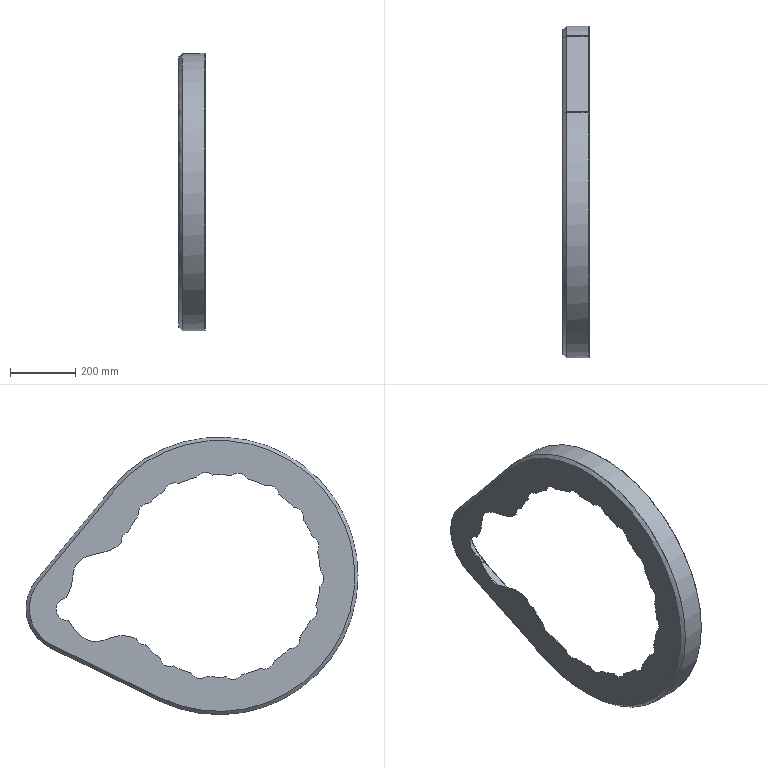Component | SolidWorks | ProtectiveCoverII-1 | 1 solid | 70 faces | volume 998867 mm3 | cylinder 46 | plane 13 | cone 9 | spline 2 | commonest cylinder face diameters 61.909 x21 620 x15 200 x3 70 x2 270 x2 850 x1 846 x1 266 x1